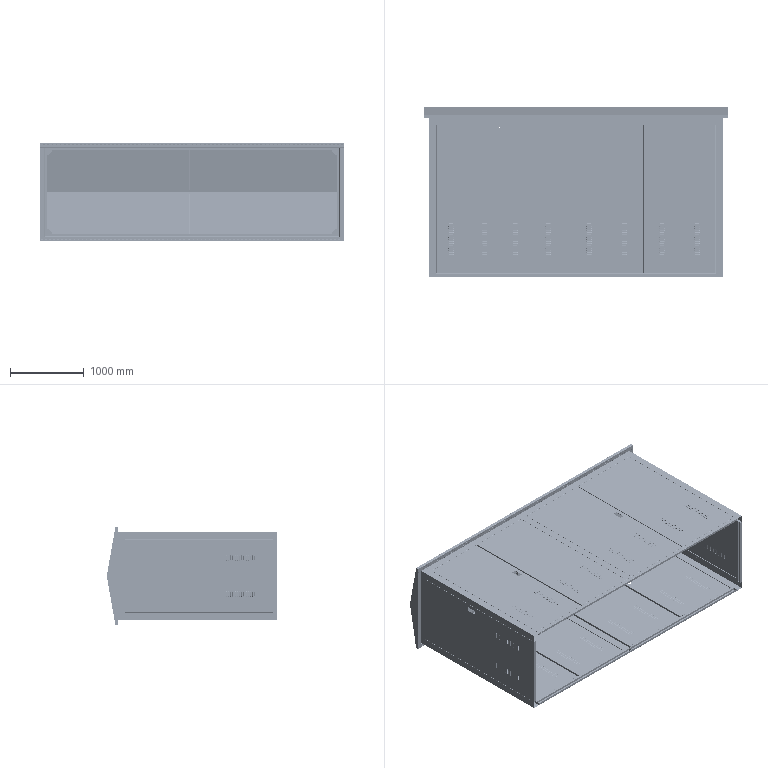Assembly | SolidWorks | mm | 41 component files | 41 solids | 12540 faces | box 4130 x 2318.76 x 1330.4 mm | volume 54133337 mm3 | cylinder 5644 | plane 4496 | torus 2400 | commonest cylinder face diameters 8 x1800 11 x1494 5 x900 6 x772 3.4 x267 0.4 x267 7 x62 9 x60
Bill of materials:
Stiffener | 4 |  | Flat plate of constant thickness. Its outline is a rectangle with one corner cut off at an angle (a chamfered pentagon) and small corner radii. It has seven round through-holes in an L-shaped pattern: three along the top edge, three down the left edge sharing the top-left hole, plus one more hole near the angled edge.
TopCover2 | 2 |  | Long, thin, formed sheet panel. Seen end-on, it is a tall straight web that leans slightly off vertical. At the top is a short stepped hook or offset flange. The top band carries many small slots in staggered rows, plus a row of small round and oblong holes just below it. The rest of the face is plain.
TopCoverOne | 2 |  | Long, thin, formed sheet panel. Its end profile is the same as unnamed part: a slightly inclined web with a stepped hook flange at the top. The top band has many small staggered slots, and below it is a row of small oblong holes that appear paired.
TopPlateSideSealingPlate | 2 |  | Formed sheet part. Its cross-section is a long straight web, a short return leg, and a stepped offset flange (Z/step-shaped). Seen from the side, the main web tapers to a central point, giving a chevron or triangular outline. The flange strips carry columns of small slots and a few larger oblong holes.
WaterproofSlot | 1 |  | Long, slender formed strip or rail. Its cross-section is a symmetric zigzag (omega-like) profile of inclined segments joined by bends with rounded corners. Faint marks spaced along its length may be small features or segment boundaries.
WaterproofSlot2 | 2 |  | Long hat-shaped or channel-type formed profile: a central channel with two side flanges. At one end the central channel extends beyond the flanges. Each flange has four small holes evenly spaced along it (8 in total).
Column | 4 |  | Long formed profile with a stepped, Z/hook-like open cross-section: a large rectangular top run, with stepped return flanges at both ends ending in short lips. Small round holes are visible near the ends of the part.
FrontDoorPanel1 | 2 |  | Large, thin rectangular flat panel. It has two groups of parallel louver or vent slots near one end, a single rectangular cutout near one long edge, and small tabs or bumps along an edge.
FrontDoorPanel2 | 2 |  | Large, thin rectangular panel similar to unnamed part. It has two arrays of parallel vent slots but no rectangular cutout. Along one long edge is a narrow bent-down flange or lip, and the other edges have small tabs or notches.
LowerCrossbeam | 1 |  | Long formed rail. Its open cross-section is a rectangular box-like portion plus a lateral U/L-shaped return flange. Each end face has two large round holes, and one face has small round holes spaced along the length. One flange is slightly shorter than the main body.
LowerCrossbeam1111111234 | 1 |  | Long formed rail similar to unnamed part. It has a rectangular section with two large round holes at the end and a lateral return flange, but the flange is oriented to the opposite side (upper) of the section. Small holes run along its length and appear on the end faces.
LowerCrossbeam1234 | 1 |  | Long formed rail with the same open profile as unnamed part: a rectangular portion plus a U-shaped side flange. Unlike that part, it shows no large holes in the end view. Small round holes are spaced along one side, and the flange is offset or shorter at one end.
LowerCrossbeam20001234 | 1 |  | Long, slender formed sheet-metal rail. Its cross-section is a U-channel with rounded bottom corners, plus a flat offset flange off the top of one side that ends in a short downturned lip.
MiddleColumn | 2 |  | Long formed rail with a hat-type cross-section: a raised central rectangular channel with a flat flange on each side, and each flange ends in a short upturned lip.
SideDoorPanel | 2 |  | Thin, flat rectangular sheet panel with two parallel rows of narrow slots (louvers) toward one end and a single rectangular cutout near one long edge.
SideLowerCrossbeam | 2 |  | Long, straight formed sheet-metal profile with a stepped, Z-like multi-bend cross-section: short top flange, vertical web, horizontal step, a longer second web, and a bottom flange.
SideUpperCrossbeam | 2 |  | Long, straight formed sheet-metal profile with a stepped cross-section: top flange, long vertical web, horizontal step, short vertical segment, and a short bottom lip.
SmallDoorPanel1 | 2 |  | Flat, rectangular, tray-like sheet panel with a shallow turned edge around the perimeter, two rows of slots (louvers) near one end, and one rectangular cutout.
SmallDoorPanel2 | 2 |  | Flat, rectangular, tray-like sheet panel with a shallow perimeter edge and two rows of slots (louvers) near one end. It has no large rectangular cutout.
UpperCrossbeam000000 | 1 |  | Long formed sheet-metal rail with a U-channel cross-section and an offset flange off the top of one side that ends in a downturned lip.
UpperCrossbeam | 1 |  | Long formed rail whose cross-section is a rectangular channel, closed on top with rounded top corners. A flat flange extends to one side at the base and ends in a short upturned lip.
UpperCrossbeam123 | 1 |  | Long formed rail with a rectangular channel section (rounded top corners) and a side base flange ending in an upturned lip. It is similar to the previous rail but has round holes in the end wall.
UpperCrossbeam20001234 | 1 |  | Long formed sheet-metal rail with a U-channel cross-section and an offset top side flange that ends in a downturned lip. It is similar to the earlier slotted U-channel rail but has obround holes in the end wall.
Mates:
1. coincident | Column-1 face at (-56.529, 19.344, 66.75) dir (0, 0, 1) | UpperCrossbeam-1 face at (880.971, 1055.344, 66.75) dir (0, 0, 1)
2. coincident | Column-1 face at (-6.529, 1105.344, 36.75) dir (0, 1, 0) | UpperCrossbeam-1 face at (880.971, 1105.344, 66.75) dir (0, 1, 0)
3. coincident | Column-1 face at (-6.529, 19.344, 66.75) dir (1, 0, 0) | UpperCrossbeam-1 face at (-6.529, 1055.344, 66.75) dir (-1, 0, 0)
4. coincident | Column-1 face at (-56.529, 19.344, 66.75) dir (0, 0, 1) | LowerCrossbeam-1 face at (880.971, -1041.656, 66.75) dir (0, 0, 1)
5. coincident | Column-1 face at (-6.529, 19.344, 66.75) dir (1, 0, 0) | LowerCrossbeam-1 face at (-6.529, -1041.656, 66.75) dir (-1, 0, 0)
6. coincident | Column-1 face at (-6.529, -1066.656, 65.25) dir (0, -1, 0) | LowerCrossbeam-1 face at (880.971, -1066.656, 66.75) dir (0, -1, 0)
7. coincident | UpperCrossbeam-1 face at (880.971, 1005.344, 66.75) dir (0, -1, 0) | MiddleColumn-1 face at (1768.471, 1005.344, 66.75) dir (0, 1, 0)
8. coincident | UpperCrossbeam-1 face at (1684.971, 971.844, 46.75) dir (1, 0, 0) | MiddleColumn-1 face at (1684.971, -5.656, 66.75) dir (-1, 0, 0)
9. coincident | UpperCrossbeam-1 face at (880.971, 1055.344, 66.75) dir (0, 0, 1) | MiddleColumn-1 face at (1768.471, -5.656, 66.75) dir (0, 0, 1)
10. coincident | UpperCrossbeam-1 face at (1768.471, 1055.344, 66.75) dir (1, 0, 0) | UpperCrossbeam123-1 face at (1768.471, 1055.344, 66.75) dir (-1, 0, 0)
11. coincident | UpperCrossbeam-1 face at (880.971, 1055.344, 66.75) dir (0, 0, 1) | UpperCrossbeam123-1 face at (2780.971, 1055.344, 66.75) dir (0, 0, 1)
12. coincident | UpperCrossbeam-1 face at (880.971, 1105.344, 66.75) dir (0, 1, 0) | UpperCrossbeam123-1 face at (2780.971, 1105.344, 66.75) dir (0, 1, 0)
13. coincident | UpperCrossbeam123-1 face at (2780.971, 1055.344, 66.75) dir (0, 0, 1) | Column-2 face at (3893.471, 19.344, 66.75) dir (0, 0, 1)
14. coincident | UpperCrossbeam123-1 face at (3793.471, 1055.344, 66.75) dir (1, 0, 0) | Column-2 face at (3793.471, 19.344, 16.75) dir (-1, 0, 0)
15. coincident | UpperCrossbeam123-1 face at (2780.971, 1105.344, 66.75) dir (0, 1, 0) | Column-2 edge at (3891.971, 1105.344, -31.55) dir (0, 0, 1)
16. coincident | LowerCrossbeam-1 face at (1768.471, -1041.656, 66.75) dir (1, 0, 0) | LowerCrossbeam1234-1 face at (1768.471, -1041.656, 66.75) dir (-1, 0, 0)
17. coincident | LowerCrossbeam-1 face at (880.971, -1041.656, 66.75) dir (0, 0, 1) | LowerCrossbeam1234-1 face at (2780.971, -1041.656, 66.75) dir (0, 0, 1)
18. coincident | LowerCrossbeam-1 face at (880.971, -1066.656, 66.75) dir (0, -1, 0) | LowerCrossbeam1234-1 face at (2780.971, -1066.656, 66.75) dir (0, -1, 0)
19. coincident | Column-2 face at (3893.471, 19.344, 16.75) dir (1, 0, 0) | SideUpperCrossbeam-1 face at (3893.471, 1055.344, -533.25) dir (1, 0, 0)
20. coincident | UpperCrossbeam123-1 face at (2780.971, 1105.344, 66.75) dir (0, 1, 0) | SideUpperCrossbeam-1 face at (3893.471, 1105.344, -533.25) dir (0, 1, 0)
21. coincident | Column-2 face at (3893.471, 19.344, -33.25) dir (0, 0, -1) | SideUpperCrossbeam-1 face at (3891.971, 1105.344, -33.25) dir (0, 0, 1)
22. coincident | Column-2 face at (3893.471, 19.344, 16.75) dir (1, 0, 0) | SideLowerCrossbeam-1 face at (3893.471, -1041.656, -533.25) dir (1, 0, 0)
23. coincident | LowerCrossbeam1234-1 face at (2780.971, -1066.656, 66.75) dir (0, -1, 0) | SideLowerCrossbeam-1 face at (3893.471, -1066.656, -533.25) dir (0, -1, 0)
24. coincident | Column-2 face at (3893.471, 19.344, -33.25) dir (0, 0, -1) | SideLowerCrossbeam-1 face at (3891.971, -1066.656, -33.25) dir (0, 0, 1)
25. coincident | SideUpperCrossbeam-1 face at (3893.471, 1055.344, -533.25) dir (1, 0, 0) | Column-3 face at (3893.471, 19.344, -1133.25) dir (1, 0, 0)
26. coincident | SideUpperCrossbeam-1 face at (3891.971, 1105.344, -1033.25) dir (0, 0, -1) | Column-3 face at (3843.471, 19.344, -1033.25) dir (0, 0, 1)
27. coincident | SideUpperCrossbeam-1 face at (3893.471, 1105.344, -533.25) dir (0, 1, 0) | Column-3 face at (3893.471, 1105.344, -1033.25) dir (0, 1, 0)
28. coincident | Column-3 face at (3843.471, 19.344, -1133.25) dir (0, 0, -1) | UpperCrossbeam000000-1 face at (2780.971, 1055.344, -1133.25) dir (0, 0, -1)
29. coincident | Column-3 face at (3793.471, 19.344, -1133.25) dir (-1, 0, 0) | UpperCrossbeam000000-1 face at (3793.471, 1055.344, -1133.25) dir (1, 0, 0)
30. coincident | SideUpperCrossbeam-1 face at (3893.471, 1105.344, -533.25) dir (0, 1, 0) | UpperCrossbeam000000-1 face at (2780.971, 1105.344, -1133.25) dir (0, 1, 0)
31. coincident | UpperCrossbeam000000-1 face at (2780.971, 1055.344, -1133.25) dir (0, 0, -1) | MiddleColumn-2 face at (1768.471, -5.656, -1133.25) dir (0, 0, -1)
32. coincident | UpperCrossbeam000000-1 face at (2780.971, 1005.344, -1133.25) dir (0, -1, 0) | MiddleColumn-2 face at (1768.471, 1005.344, -1133.25) dir (0, 1, 0)
33. coincident | UpperCrossbeam000000-1 face at (1851.971, 1005.344, -1103.25) dir (-1, 0, 0) | MiddleColumn-2 face at (1851.971, -5.656, -1133.25) dir (1, 0, 0)
34. coincident | Column-3 face at (3843.471, 19.344, -1133.25) dir (0, 0, -1) | LowerCrossbeam20001234-1 face at (2780.971, -1041.656, -1133.25) dir (0, 0, -1)
35. coincident | Column-3 face at (3793.471, 19.344, -1133.25) dir (-1, 0, 0) | LowerCrossbeam20001234-1 face at (3793.471, -1041.656, -1133.25) dir (1, 0, 0)
36. coincident | SideLowerCrossbeam-1 face at (3893.471, -1066.656, -533.25) dir (0, -1, 0) | LowerCrossbeam20001234-1 face at (2780.971, -1066.656, -1133.25) dir (0, -1, 0)
37. coincident | UpperCrossbeam000000-1 face at (1768.471, 1055.344, -1133.25) dir (-1, 0, 0) | UpperCrossbeam20001234-2 face at (1768.471, 1055.344, -1133.25) dir (1, 0, 0)
38. coincident | UpperCrossbeam000000-1 face at (2780.971, 1105.344, -1133.25) dir (0, 1, 0) | UpperCrossbeam20001234-2 face at (880.971, 1105.344, -1133.25) dir (0, 1, 0)
39. coincident | UpperCrossbeam000000-1 face at (2780.971, 1055.344, -1133.25) dir (0, 0, -1) | UpperCrossbeam20001234-2 face at (880.971, 1055.344, -1133.25) dir (0, 0, -1)
40. coincident | UpperCrossbeam20001234-2 face at (880.971, 1055.344, -1133.25) dir (0, 0, -1) | Column-4 face at (-106.529, 19.344, -1133.25) dir (0, 0, -1)
41. coincident | UpperCrossbeam20001234-2 face at (880.971, 1105.344, -1133.25) dir (0, 1, 0) | Column-4 face at (-105.029, 1105.344, -1133.25) dir (0, 1, 0)
42. coincident | UpperCrossbeam20001234-2 face at (-6.529, 1055.344, -1133.25) dir (-1, 0, 0) | Column-4 face at (-6.529, 19.344, -1083.25) dir (1, 0, 0)
43. coincident | MiddleColumn-2 face at (1768.471, -5.656, -1133.25) dir (0, 0, -1) | LowerCrossbeam1111111234-1 face at (880.971, -1041.656, -1133.25) dir (0, 0, -1)
44. coincident | MiddleColumn-2 face at (1768.471, -1016.656, -1133.25) dir (0, -1, 0) | LowerCrossbeam1111111234-1 face at (880.971, -1016.656, -1133.25) dir (0, 1, 0)
45. coincident | LowerCrossbeam20001234-1 face at (1768.471, -1041.656, -1133.25) dir (-1, 0, 0) | LowerCrossbeam1111111234-1 face at (1768.471, -1041.656, -1133.25) dir (1, 0, 0)
46. coincident | Column-4 face at (-106.529, 19.344, -1083.25) dir (-1, 0, 0) | SideUpperCrossbeam-2 face at (-106.529, 1055.344, -533.25) dir (-1, 0, 0)
47. coincident | Column-4 face at (-6.529, 1105.344, -1133.25) dir (0, 1, 0) | SideUpperCrossbeam-2 face at (-106.529, 1105.344, -533.25) dir (0, 1, 0)
48. coincident | Column-4 face at (-106.529, 19.344, -1033.25) dir (0, 0, 1) | SideUpperCrossbeam-2 face at (-105.029, 1105.344, -1033.25) dir (0, 0, -1)
49. coincident | Column-4 face at (-106.529, 19.344, -1083.25) dir (-1, 0, 0) | SideLowerCrossbeam-2 face at (-106.529, -1041.656, -533.25) dir (-1, 0, 0)
50. coincident | Column-4 face at (-106.529, 19.344, -1033.25) dir (0, 0, 1) | SideLowerCrossbeam-2 face at (-105.029, -1066.656, -1033.25) dir (0, 0, -1)
51. coincident | LowerCrossbeam1111111234-1 face at (880.971, -1066.656, -1133.25) dir (0, -1, 0) | SideLowerCrossbeam-2 face at (-106.529, -1066.656, -533.25) dir (0, -1, 0)
52. coincident | UpperCrossbeam-1 face at (880.971, 1105.344, 66.75) dir (0, 1, 0) | Assembly2-1/TopCover2-1 face at (832.971, 1105.344, -200.589) dir (0, -1, 0)
53. distance | Assembly2-1/TopPlateSideSealingPlate-2 face at (-111.529, 1094.844, -533.606) dir (1, 0, 0) | Column-1 face at (-106.529, 19.344, 66.75) dir (-1, 0, 0)
54. distance | Assembly2-1/TopCover2-1 face at (832.971, 1193.444, 71.75) dir (0, 0, -1) | Column-1 face at (-56.529, 19.344, 66.75) dir (0, 0, 1)
55. distance | FrontDoorPanel1-1 face at (2310.971, 1002.844, 66.75) dir (0, 1, 0) | UpperCrossbeam-1 face at (880.971, 1005.344, 66.75) dir (0, -1, 0)
56. distance | FrontDoorPanel1-1 face at (1820.971, -5.656, 66.75) dir (-1, 0, 0) | MiddleColumn-1 face at (1818.471, -5.656, 66.75) dir (1, 0, 0)
57. coincident | FrontDoorPanel1-1 face at (2310.971, -5.656, 66.75) dir (0, 0, 1) | FrontDoorPanel2-1 face at (3300.971, -5.656, 66.75) dir (0, 0, 1)
58. distance | FrontDoorPanel2-1 face at (3300.971, -1014.156, 66.75) dir (0, -1, 0) | LowerCrossbeam1234-1 face at (2780.971, -1016.656, 66.75) dir (0, 1, 0)
59. coincident | MiddleColumn-2 face at (1768.471, -5.656, -1133.25) dir (0, 0, -1) | FrontDoorPanel2-2 face at (2310.971, -5.656, -1133.25) dir (0, 0, -1)
60. distance | FrontDoorPanel2-2 face at (1820.971, -5.656, -1133.25) dir (-1, 0, 0) | MiddleColumn-2 face at (1818.471, -5.656, -1133.25) dir (1, 0, 0)
61. distance | FrontDoorPanel2-2 face at (2310.971, -1014.156, -1133.25) dir (0, -1, 0) | LowerCrossbeam20001234-1 face at (2780.971, -1016.656, -1133.25) dir (0, 1, 0)
62. coincident | FrontDoorPanel2-2 face at (2310.971, -5.656, -1133.25) dir (0, 0, -1) | FrontDoorPanel1-2 face at (3300.971, -5.656, -1133.25) dir (0, 0, -1)
63. distance | FrontDoorPanel1-2 face at (3300.971, 1002.844, -1133.25) dir (0, 1, 0) | UpperCrossbeam000000-1 face at (2780.971, 1005.344, -1133.25) dir (0, -1, 0)
64. distance | FrontDoorPanel1-2 face at (3790.971, -5.656, -1133.25) dir (1, 0, 0) | Column-3 face at (3793.471, 19.344, -1133.25) dir (-1, 0, 0)
65. coincident | FrontDoorPanel2-2 face at (2310.971, -5.656, -1133.25) dir (0, 0, -1) | SmallDoorPanel1-1 face at (1288.471, -5.656, -1133.25) dir (0, 0, -1)
66. distance | SmallDoorPanel1-1 face at (1288.471, -1014.156, -1133.25) dir (0, -1, 0) | LowerCrossbeam1111111234-1 face at (880.971, -1016.656, -1133.25) dir (0, 1, 0)
67. coincident | FrontDoorPanel2-2 face at (2310.971, -5.656, -1133.25) dir (0, 0, -1) | SmallDoorPanel1-1 face at (1288.471, -5.656, -1133.25) dir (0, 0, -1)
68. distance | SmallDoorPanel1-1 face at (1715.971, -5.656, -1133.25) dir (1, 0, 0) | MiddleColumn-2 face at (1718.471, -5.656, -1133.25) dir (-1, 0, 0)
69. coincident | Column-4 face at (-106.529, 19.344, -1133.25) dir (0, 0, -1) | SmallDoorPanel2-1 face at (419.721, -5.656, -1133.25) dir (0, 0, -1)
70. distance | SmallDoorPanel2-1 face at (-4.029, -5.656, -1133.25) dir (-1, 0, 0) | Column-4 face at (-6.529, 19.344, -1083.25) dir (1, 0, 0)
71. coincident | SmallDoorPanel1-1 face at (1288.471, 1002.844, -1133.25) dir (0, 1, 0) | SmallDoorPanel2-1 face at (419.721, 1002.844, -1133.25) dir (0, 1, 0)
72. coincident | Column-3 face at (3893.471, 19.344, -1133.25) dir (1, 0, 0) | SideDoorPanel-1 face at (3893.471, -5.656, -533.25) dir (1, 0, 0)
73. distance | SideDoorPanel-1 face at (3891.971, -5.656, -35.75) dir (0, 0, 1) | Column-2 face at (3893.471, 19.344, -33.25) dir (0, 0, -1)
74. distance | SideDoorPanel-1 face at (3891.971, 1002.844, -533.25) dir (0, 1, 0) | SideUpperCrossbeam-1 face at (3893.471, 1005.344, -533.25) dir (0, -1, 0)
75. coincident | Column-1 face at (-106.529, 19.344, 66.75) dir (-1, 0, 0) | SideDoorPanel-2 face at (-106.529, -5.656, -533.25) dir (-1, 0, 0)
76. distance | SideDoorPanel-2 face at (-105.029, -5.656, -1030.75) dir (0, 0, -1) | Column-4 face at (-106.529, 19.344, -1033.25) dir (0, 0, 1)
77. distance | SideDoorPanel-2 face at (-105.029, 1002.844, -533.25) dir (0, 1, 0) | SideUpperCrossbeam-2 face at (-106.529, 1005.344, -533.25) dir (0, -1, 0)
78. coincident | Column-1 face at (-56.529, 19.344, 66.75) dir (0, 0, 1) | SmallDoorPanel1-2 face at (423.471, -5.656, 66.75) dir (0, 0, 1)
79. distance | SmallDoorPanel1-2 face at (-4.029, -5.656, 66.75) dir (-1, 0, 0) | Column-1 face at (-6.529, 19.344, 66.75) dir (1, 0, 0)
80. distance | SmallDoorPanel1-2 face at (423.471, -1014.156, 66.75) dir (0, -1, 0) | LowerCrossbeam-1 face at (880.971, -1016.656, 66.75) dir (0, 1, 0)
81. coincident | FrontDoorPanel1-1 face at (2310.971, -5.656, 66.75) dir (0, 0, 1) | SmallDoorPanel2-2 face at (1292.221, -5.656, 66.75) dir (0, 0, 1)
82. distance | SmallDoorPanel2-2 face at (1715.971, -5.656, 66.75) dir (1, 0, 0) | MiddleColumn-1 face at (1718.471, -5.656, 66.75) dir (-1, 0, 0)
83. distance | SmallDoorPanel2-2 face at (1292.221, 1002.844, 66.75) dir (0, 1, 0) | UpperCrossbeam-1 face at (880.971, 1005.344, 66.75) dir (0, -1, 0)
84. distance | Column-2 face at (3793.471, 19.344, 16.75) dir (-1, 0, 0) | FrontDoorPanel2-1 face at (3790.971, -5.656, 66.75) dir (1, 0, 0)
85. coincident | Column-2 face at (3893.471, 19.344, 66.75) dir (0, 0, 1) | FrontDoorPanel2-1 face at (3300.971, -5.656, 66.75) dir (0, 0, 1)
86. coincident | TopCover2-1 face at (929.837, -331.061, 23.271) dir (1, 0, 0) | TopCover2-2 face at (929.837, 979.123, -207.75) dir (1, 0, 0)
87. coincident | TopCover2-1 face at (-73.163, -10.453, -72.331) dir (0, -0.1736, -0.9848) | TopCover2-2 face at (-73.163, 645.152, -187.932) dir (0, -0.1736, -0.9848)
88. coincident | TopCover2-1 face at (-73.163, 334.425, -33.29) dir (0, 0.9848, -0.1736) | TopCover2-2 face at (-73.163, 334.425, -33.29) dir (0, -0.9848, 0.1736)
89. coincident | TopCover2-1 face at (-73.163, 6.669, 24.771) dir (0, 0, 1) | TopCoverOne-1 face at (1990.337, 6.669, 24.771) dir (0, 0, 1)
90. coincident | TopCover2-1 face at (-73.163, -320.575, 82.741) dir (0, -0.9848, 0.1736) | TopCoverOne-1 face at (1990.337, -320.575, 82.741) dir (0, -0.9848, 0.1736)
91. coincident | TopCover2-1 face at (929.837, -276.57, -13.223) dir (1, 0, 0) | TopCoverOne-1 face at (929.837, -242.102, -19.3) dir (-1, 0, 0)
92. coincident | TopCoverOne-1 face at (1990.337, 334.425, -33.29) dir (0, 0.9848, -0.1736) | TopCoverOne-2 face at (1990.337, 334.425, -33.29) dir (0, -0.9848, 0.1736)
93. coincident | TopCover2-2 face at (-73.163, 645.152, -187.932) dir (0, -0.1736, -0.9848) | TopCoverOne-2 face at (1990.337, 645.152, -187.932) dir (0, -0.1736, -0.9848)
94. coincident | TopCover2-2 edge at (929.837, 346.567, 24.078) dir (0, 0.9397, -0.342) | TopCoverOne-2 face at (929.837, 979.123, -207.75) dir (-1, 0, 0)
95. coincident | TopCoverOne-2 face at (3050.837, 880.969, -217.328) dir (1, 0, 0) | TopPlateSideSealingPlate-1 face at (3050.837, 317.506, -130.159) dir (-1, 0, 0)
96. coincident | TopCoverOne-2 face at (1990.337, 645.152, -187.932) dir (0, -0.1736, -0.9848) | TopPlateSideSealingPlate-1 face at (3052.337, 317.506, -130.159) dir (0, -0.1736, -0.9848)
97. coincident | TopCoverOne-2 face at (1990.337, 989.61, -148.28) dir (0, 0.9848, -0.1736) | TopPlateSideSealingPlate-1 face at (3050.837, 972.442, -245.642) dir (0, 0.9848, -0.1736)
98. coincident | TopCover2-1 face at (-73.163, -10.453, -72.331) dir (0, -0.1736, -0.9848) | TopPlateSideSealingPlate-2 face at (-1077.663, 317.506, -130.159) dir (0, -0.1736, -0.9848)
99. coincident | TopCover2-2 face at (-1076.163, 979.123, -207.75) dir (-1, 0, 0) | TopPlateSideSealingPlate-2 face at (-1076.163, 317.506, -130.159) dir (1, 0, 0)
100. coincident | TopCover2-2 face at (-73.163, 989.61, -148.28) dir (0, 0.9848, -0.1736) | TopPlateSideSealingPlate-2 face at (-1076.163, 972.442, -245.642) dir (0, 0.9848, -0.1736)
101. distance | WaterproofSlot-1 face at (-1061.163, 371.107, 13.55) dir (-1, 0, 0) | TopPlateSideSealingPlate-2 face at (-1076.163, 317.506, -130.159) dir (1, 0, 0)
102. coincident | TopCoverOne-1 face at (1990.337, 6.669, 23.271) dir (0, 0, -1) | WaterproofSlot-1 face at (988.837, 340.977, 23.271) dir (0, 0, 1)
103. coincident | TopCoverOne-2 face at (1990.337, 661.761, -92.24) dir (0, -0.342, -0.9397) | WaterproofSlot-1 edge at (3038.837, 383.793, 8.933) dir (-1, 0, 0)
104. coincident | TopCover2-1 face at (-73.163, -8.63, -61.991) dir (0, -0.1736, -0.9848) | Stiffener-2 face at (-916.663, -223.482, -24.107) dir (0, 0.1736, 0.9848)
105. distance | Stiffener-2 face at (-1008.663, -270.285, -17.885) dir (0, -0.9848, 0.1736) | TopCover2-1 face at (-73.163, -261.533, 72.062) dir (0, 0.9848, -0.1736)
106. distance | Stiffener-2 face at (-1010.663, -268.315, -18.232) dir (-1, 0, 0) | TopPlateSideSealingPlate-2 face at (-1017.663, 317.506, -130.159) dir (1, 0, 0)
107. coincident | Stiffener-2 face at (-916.663, -223.83, -26.076) dir (0, -0.1736, -0.9848) | Stiffener-3 face at (-963.491, 815.364, -209.314) dir (0, -0.1736, -0.9848)
108. distance | Stiffener-3 face at (-1010.663, 905.966, -225.29) dir (-1, 0, 0) | TopPlateSideSealingPlate-2 face at (-1017.663, 317.506, -130.159) dir (1, 0, 0)
109. distance | Stiffener-3 face at (-1008.663, 907.936, -225.637) dir (0, 0.9848, -0.1736) | TopCover2-2 face at (-73.163, 930.475, -138.121) dir (0, -0.9848, 0.1736)
110. coincident | Stiffener-3 face at (-963.491, 815.364, -209.314) dir (0, -0.1736, -0.9848) | Stiffener-4 face at (2938.166, 815.364, -209.314) dir (0, -0.1736, -0.9848)
111. distance | Stiffener-4 face at (2985.337, 906.314, -223.32) dir (1, 0, 0) | TopPlateSideSealingPlate-1 face at (2992.337, 317.506, -130.159) dir (-1, 0, 0)
112. distance | Stiffener-4 face at (2983.337, 908.283, -223.667) dir (0, 0.9848, -0.1736) | TopCoverOne-2 face at (1990.337, 930.475, -138.121) dir (0, -0.9848, 0.1736)
113. coincident | Stiffener-4 face at (2938.166, 815.364, -209.314) dir (0, -0.1736, -0.9848) | Stiffener-5 face at (2938.166, -177.713, -34.208) dir (0, -0.1736, -0.9848)
114. distance | Stiffener-5 face at (2983.337, -270.285, -17.885) dir (0, -0.9848, 0.1736) | TopCoverOne-1 face at (1990.337, -261.533, 72.062) dir (0, 0.9848, -0.1736)
115. distance | Stiffener-5 face at (2985.337, -268.315, -18.232) dir (1, 0, 0) | TopPlateSideSealingPlate-1 face at (2992.337, 317.506, -130.159) dir (-1, 0, 0)
116. coincident | TopCover2-1 face at (-73.163, 6.669, 23.271) dir (0, 0, -1) | WaterproofSlot2-1 face at (929.837, -4.023, 23.271) dir (0, 0, 1)
117. coincident | WaterproofSlot-1 face at (988.837, 315.977, 4.771) dir (0, -1, 0) | WaterproofSlot2-1 face at (954.837, 315.977, 4.771) dir (0, 1, 0)
118. distance | WaterproofSlot2-1 face at (904.837, -4.023, 4.771) dir (-1, 0, 0) | TopCover2-2 edge at (929.837, 346.054, 22.668) dir (0, 0.9397, -0.342)
119. coincident | TopCoverOne-2 face at (1990.337, 661.761, -92.24) dir (0, -0.342, -0.9397) | WaterproofSlot2-2 edge at (891.337, 972.51, -205.343) dir (0, -0.9397, 0.342)
120. coincident | WaterproofSlot-1 face at (988.837, 364.779, -3.834) dir (0, 0.9397, -0.342) | WaterproofSlot2-2 face at (954.837, 364.779, -3.834) dir (0, -0.9397, 0.342)
121. coincident | WaterproofSlot2-1 face at (904.837, -4.023, 4.771) dir (-1, 0, 0) | WaterproofSlot2-2 face at (904.837, 665.481, -113.281) dir (-1, 0, 0)